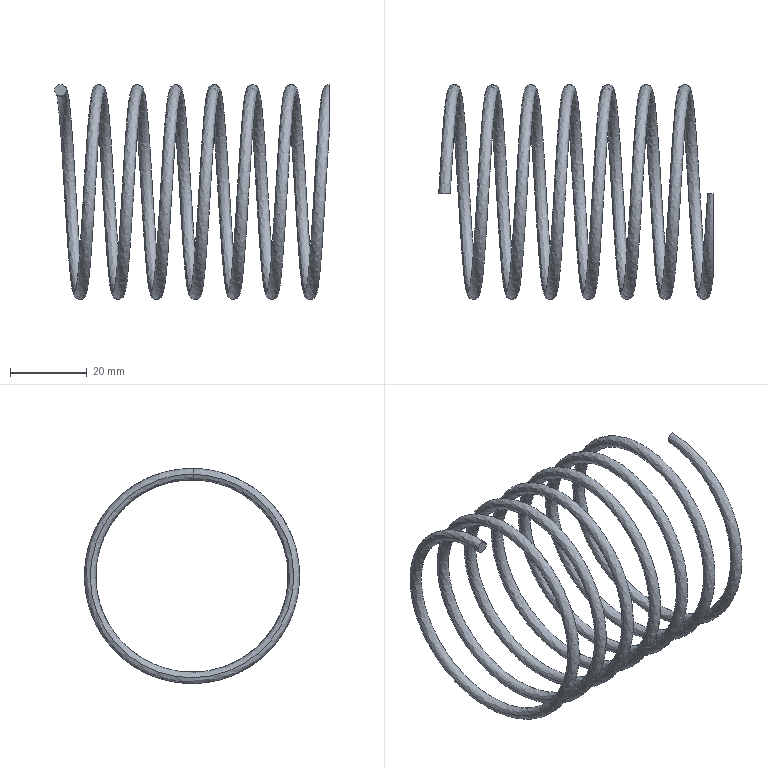Component | SolidWorks | 216InnerTubeAssembly-1_CompressionRecoverySpring-1 | 1 solid | 5 faces | volume 8195 mm3 | plane 3 | spline 2